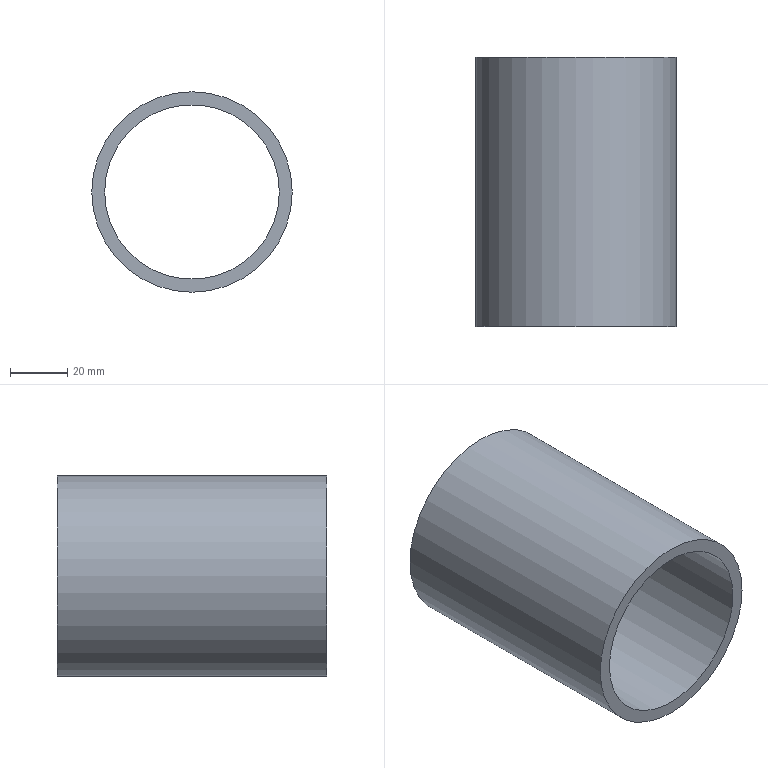Component | NX | SPACER_SLEEVE | 1 solid | 4 faces | box 70 x 94 x 70 mm | volume 87043 mm3 | cylinder 2 | plane 2 | commonest cylinder face diameters 70 x1 61 x1
STEP:
#1=CARTESIAN_POINT('',(0.,0.,0.));
#2=DIRECTION('',(0.,0.,1.));
#3=DIRECTION('',(1.,0.,0.));
#4=AXIS2_PLACEMENT_3D('',#1,#2,#3);
#5=CARTESIAN_POINT('',(32.,-74.5,-3.));
#6=VERTEX_POINT('',#5);
#7=CARTESIAN_POINT('',(-3.,-74.5,-3.));
#8=DIRECTION('',(0.,-1.,0.));
#9=DIRECTION('',(1.,0.,-0.));
#10=AXIS2_PLACEMENT_3D('',#7,#8,#9);
#11=CIRCLE('',#10,35.);
#12=CARTESIAN_POINT('',(-3.,-74.5,-3.));
#13=DIRECTION('',(0.,1.,0.));
#14=DIRECTION('',(0.,0.,1.));
#15=AXIS2_PLACEMENT_3D('',#12,#13,#14);
#16=CYLINDRICAL_SURFACE('',#15,35.);
#17=CARTESIAN_POINT('',(7.854,0.));
#18=DIRECTION('',(-1.,0.));
#19=VECTOR('',#18,1.);
#20=LINE('',#17,#19);
#21=(GEOMETRIC_REPRESENTATION_CONTEXT(2)PARAMETRIC_REPRESENTATION_CONTEXT()REPRESENTATION_CONTEXT('',''));
#22=DEFINITIONAL_REPRESENTATION('',(#20),#21);
#23=PCURVE('',#16,#22);
#24=CARTESIAN_POINT('',(-3.,-74.5,-3.));
#25=DIRECTION('',(0.,-1.,0.));
#26=DIRECTION('',(0.,0.,-1.));
#27=AXIS2_PLACEMENT_3D('',#24,#25,#26);
#28=PLANE('',#27);
#29=CARTESIAN_POINT('',(0.,0.));
#30=DIRECTION('',(0.,1.));
#31=AXIS2_PLACEMENT_2D('',#29,#30);
#32=CIRCLE('',#31,35.);
#33=(GEOMETRIC_REPRESENTATION_CONTEXT(2)PARAMETRIC_REPRESENTATION_CONTEXT()REPRESENTATION_CONTEXT('',''));
#34=DEFINITIONAL_REPRESENTATION('',(#32),#33);
#35=PCURVE('',#28,#34);
#36=SURFACE_CURVE('',#11,(#23,#35),.PCURVE_S1.);
#37=EDGE_CURVE('',#6,#6,#36,.T.);
#38=ORIENTED_EDGE('',*,*,#37,.F.);
#39=CARTESIAN_POINT('',(32.,19.5,-3.));
#40=VERTEX_POINT('',#39);
#41=CARTESIAN_POINT('',(32.,-74.5,-3.));
#42=CARTESIAN_POINT('',(32.,19.5,-3.));
#43=B_SPLINE_CURVE_WITH_KNOTS('',1,(#41,#42),.UNSPECIFIED.,.F.,.F.,(2,2),(0.,94.),.PIECEWISE_BEZIER_KNOTS.);
#44=CARTESIAN_POINT('',(7.854,0.));
#45=DIRECTION('',(0.,1.));
#46=VECTOR('',#45,1.);
#47=LINE('',#44,#46);
#48=(GEOMETRIC_REPRESENTATION_CONTEXT(2)PARAMETRIC_REPRESENTATION_CONTEXT()REPRESENTATION_CONTEXT('',''));
#49=DEFINITIONAL_REPRESENTATION('',(#47),#48);
#50=PCURVE('',#16,#49);
#51=CARTESIAN_POINT('',(1.571,0.));
#52=DIRECTION('',(0.,1.));
#53=VECTOR('',#52,1.);
#54=LINE('',#51,#53);
#55=(GEOMETRIC_REPRESENTATION_CONTEXT(2)PARAMETRIC_REPRESENTATION_CONTEXT()REPRESENTATION_CONTEXT('',''));
#56=DEFINITIONAL_REPRESENTATION('',(#54),#55);
#57=PCURVE('',#16,#56);
#58=SEAM_CURVE('',#43,(#50,#57),.PCURVE_S1.);
#59=EDGE_CURVE('',#6,#40,#58,.T.);
#60=ORIENTED_EDGE('',*,*,#59,.T.);
#61=CARTESIAN_POINT('',(-3.,19.5,-3.));
#62=DIRECTION('',(0.,-1.,0.));
#63=DIRECTION('',(1.,0.,-0.));
#64=AXIS2_PLACEMENT_3D('',#61,#62,#63);
#65=CIRCLE('',#64,35.);
#66=CARTESIAN_POINT('',(7.854,94.));
#67=DIRECTION('',(-1.,0.));
#68=VECTOR('',#67,1.);
#69=LINE('',#66,#68);
#70=(GEOMETRIC_REPRESENTATION_CONTEXT(2)PARAMETRIC_REPRESENTATION_CONTEXT()REPRESENTATION_CONTEXT('',''));
#71=DEFINITIONAL_REPRESENTATION('',(#69),#70);
#72=PCURVE('',#16,#71);
#73=CARTESIAN_POINT('',(-3.,19.5,-3.));
#74=DIRECTION('',(0.,-1.,0.));
#75=DIRECTION('',(0.,0.,-1.));
#76=AXIS2_PLACEMENT_3D('',#73,#74,#75);
#77=PLANE('',#76);
#78=CARTESIAN_POINT('',(0.,0.));
#79=DIRECTION('',(0.,1.));
#80=AXIS2_PLACEMENT_2D('',#78,#79);
#81=CIRCLE('',#80,35.);
#82=(GEOMETRIC_REPRESENTATION_CONTEXT(2)PARAMETRIC_REPRESENTATION_CONTEXT()REPRESENTATION_CONTEXT('',''));
#83=DEFINITIONAL_REPRESENTATION('',(#81),#82);
#84=PCURVE('',#77,#83);
#85=SURFACE_CURVE('',#65,(#72,#84),.PCURVE_S1.);
#86=EDGE_CURVE('',#40,#40,#85,.T.);
#87=ORIENTED_EDGE('',*,*,#86,.T.);
#88=ORIENTED_EDGE('',*,*,#59,.F.);
#89=EDGE_LOOP('',(#38,#60,#87,#88));
#90=FACE_BOUND('',#89,.T.);
#91=ADVANCED_FACE('',(#90),#16,.T.);
#92=CARTESIAN_POINT('',(27.5,-74.5,-3.));
#93=VERTEX_POINT('',#92);
#94=CARTESIAN_POINT('',(-3.,-74.5,-3.));
#95=DIRECTION('',(0.,-1.,0.));
#96=DIRECTION('',(1.,0.,-0.));
#97=AXIS2_PLACEMENT_3D('',#94,#95,#96);
#98=CIRCLE('',#97,30.5);
#99=CARTESIAN_POINT('',(-3.,-74.5,-3.));
#100=DIRECTION('',(0.,1.,0.));
#101=DIRECTION('',(0.,0.,1.));
#102=AXIS2_PLACEMENT_3D('',#99,#100,#101);
#103=CYLINDRICAL_SURFACE('',#102,30.5);
#104=CARTESIAN_POINT('',(7.854,0.));
#105=DIRECTION('',(-1.,0.));
#106=VECTOR('',#105,1.);
#107=LINE('',#104,#106);
#108=(GEOMETRIC_REPRESENTATION_CONTEXT(2)PARAMETRIC_REPRESENTATION_CONTEXT()REPRESENTATION_CONTEXT('',''));
#109=DEFINITIONAL_REPRESENTATION('',(#107),#108);
#110=PCURVE('',#103,#109);
#111=CARTESIAN_POINT('',(0.,0.));
#112=DIRECTION('',(0.,1.));
#113=AXIS2_PLACEMENT_2D('',#111,#112);
#114=CIRCLE('',#113,30.5);
#115=(GEOMETRIC_REPRESENTATION_CONTEXT(2)PARAMETRIC_REPRESENTATION_CONTEXT()REPRESENTATION_CONTEXT('',''));
#116=DEFINITIONAL_REPRESENTATION('',(#114),#115);
#117=PCURVE('',#28,#116);
#118=SURFACE_CURVE('',#98,(#110,#117),.PCURVE_S1.);
#119=EDGE_CURVE('',#93,#93,#118,.T.);
#120=ORIENTED_EDGE('',*,*,#119,.F.);
#121=CARTESIAN_POINT('',(27.5,19.5,-3.));
#122=VERTEX_POINT('',#121);
#123=CARTESIAN_POINT('',(27.5,-74.5,-3.));
#124=CARTESIAN_POINT('',(27.5,19.5,-3.));
#125=B_SPLINE_CURVE_WITH_KNOTS('',1,(#123,#124),.UNSPECIFIED.,.F.,.F.,(2,2),(0.,94.),.PIECEWISE_BEZIER_KNOTS.);
#126=CARTESIAN_POINT('',(7.854,0.));
#127=DIRECTION('',(0.,1.));
#128=VECTOR('',#127,1.);
#129=LINE('',#126,#128);
#130=(GEOMETRIC_REPRESENTATION_CONTEXT(2)PARAMETRIC_REPRESENTATION_CONTEXT()REPRESENTATION_CONTEXT('',''));
#131=DEFINITIONAL_REPRESENTATION('',(#129),#130);
#132=PCURVE('',#103,#131);
#133=CARTESIAN_POINT('',(1.571,0.));
#134=DIRECTION('',(0.,1.));
#135=VECTOR('',#134,1.);
#136=LINE('',#133,#135);
#137=(GEOMETRIC_REPRESENTATION_CONTEXT(2)PARAMETRIC_REPRESENTATION_CONTEXT()REPRESENTATION_CONTEXT('',''));
#138=DEFINITIONAL_REPRESENTATION('',(#136),#137);
#139=PCURVE('',#103,#138);
#140=SEAM_CURVE('',#125,(#132,#139),.PCURVE_S1.);
#141=EDGE_CURVE('',#93,#122,#140,.T.);
#142=ORIENTED_EDGE('',*,*,#141,.T.);
#143=CARTESIAN_POINT('',(-3.,19.5,-3.));
#144=DIRECTION('',(0.,-1.,0.));
#145=DIRECTION('',(1.,0.,-0.));
#146=AXIS2_PLACEMENT_3D('',#143,#144,#145);
#147=CIRCLE('',#146,30.5);
#148=CARTESIAN_POINT('',(7.854,94.));
#149=DIRECTION('',(-1.,0.));
#150=VECTOR('',#149,1.);
#151=LINE('',#148,#150);
#152=(GEOMETRIC_REPRESENTATION_CONTEXT(2)PARAMETRIC_REPRESENTATION_CONTEXT()REPRESENTATION_CONTEXT('',''));
#153=DEFINITIONAL_REPRESENTATION('',(#151),#152);
#154=PCURVE('',#103,#153);
#155=CARTESIAN_POINT('',(0.,0.));
#156=DIRECTION('',(0.,1.));
#157=AXIS2_PLACEMENT_2D('',#155,#156);
#158=CIRCLE('',#157,30.5);
#159=(GEOMETRIC_REPRESENTATION_CONTEXT(2)PARAMETRIC_REPRESENTATION_CONTEXT()REPRESENTATION_CONTEXT('',''));
#160=DEFINITIONAL_REPRESENTATION('',(#158),#159);
#161=PCURVE('',#77,#160);
#162=SURFACE_CURVE('',#147,(#154,#161),.PCURVE_S1.);
#163=EDGE_CURVE('',#122,#122,#162,.T.);
#164=ORIENTED_EDGE('',*,*,#163,.T.);
#165=ORIENTED_EDGE('',*,*,#141,.F.);
#166=EDGE_LOOP('',(#120,#142,#164,#165));
#167=FACE_BOUND('',#166,.F.);
#168=ADVANCED_FACE('',(#167),#103,.F.);
#169=ORIENTED_EDGE('',*,*,#37,.T.);
#170=EDGE_LOOP('',(#169));
#171=FACE_BOUND('',#170,.T.);
#172=ORIENTED_EDGE('',*,*,#119,.F.);
#173=EDGE_LOOP('',(#172));
#174=FACE_BOUND('',#173,.T.);
#175=ADVANCED_FACE('',(#171,#174),#28,.T.);
#176=ORIENTED_EDGE('',*,*,#86,.F.);
#177=EDGE_LOOP('',(#176));
#178=FACE_BOUND('',#177,.T.);
#179=ORIENTED_EDGE('',*,*,#163,.T.);
#180=EDGE_LOOP('',(#179));
#181=FACE_BOUND('',#180,.T.);
#182=ADVANCED_FACE('',(#178,#181),#77,.F.);
#183=CLOSED_SHELL('',(#91,#168,#175,#182));
#184=MANIFOLD_SOLID_BREP('',#183);
#185=(LENGTH_UNIT()NAMED_UNIT(*)SI_UNIT(.MILLI.,.METRE.));
#186=UNCERTAINTY_MEASURE_WITH_UNIT(LENGTH_MEASURE(0.00001),#185,'','');
#187=(NAMED_UNIT(*)PLANE_ANGLE_UNIT()SI_UNIT($,.RADIAN.));
#188=(NAMED_UNIT(*)SI_UNIT($,.STERADIAN.)SOLID_ANGLE_UNIT());
#189=(GEOMETRIC_REPRESENTATION_CONTEXT(3)GLOBAL_UNCERTAINTY_ASSIGNED_CONTEXT((#186))GLOBAL_UNIT_ASSIGNED_CONTEXT((#185,#187,#188))REPRESENTATION_CONTEXT('',''));
#190=ADVANCED_BREP_SHAPE_REPRESENTATION('',(#4,#184),#189);